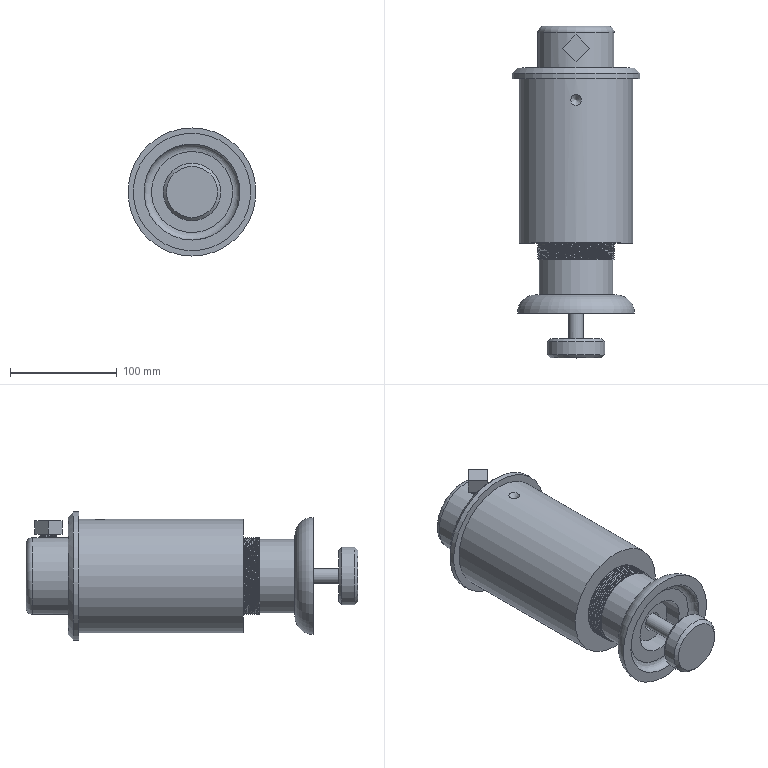Assembly | NX | mm | 5 component files | 5 solids | 128 faces | box 120 x 311 x 120 mm | volume 1746879 mm3 | cylinder 66 | plane 33 | spline 20 | cone 6 | torus 3 | commonest cylinder face diameters 14 x40 72 x4 12 x2 40 x2 45 x2 16 x2 43.5 x2 70 x2
Bill of materials:
unnamed part 1 | 1 |  | Hollow, axially symmetric flanged sleeve. A large flange with a rounded outer edge sits at one end. Next to it is a plain cylindrical section, followed by an externally threaded section that runs to the far end. A through-bore runs along the axis, and the flange face has a shallow stepped recess around the bore.
unnamed part 2 | 1 |  | Thick-walled cylindrical tube with a thin flange at one end. The flange's outer edge is chamfered. There is a small radial hole in the wall near the flange, and the bore at the non-flanged end appears to be internally threaded.
unnamed part 3 | 1 |  | Square-head bolt or screw. It has a square prismatic head and a fully threaded cylindrical shank with a chamfered tip.
unnamed part 4 | 1 |  | Stepped cylindrical shaft or body. The larger-diameter section has a rounded end, a large transverse through-hole, and a small radial hole that appears threaded near the end. The smaller-diameter section has an externally threaded band between plain sections, and an axial bore opens at the small end.
unnamed part 5 | 1 |  | Long slender screw with a short cylindrical head chamfered on both edges. A long plain unthreaded shank leads to an externally threaded section at the tip.
Mates:
1. fix | tool_holder 1 component
2. touch align | bushing 1 face | tool_holder 1 face
3. touch align | screw_sleeve 1 face | bushing 1 face
4. distance | screw_sleeve 1 face | bushing 1 face
5. distance | bushing 1 face | tool_holder 1 face
6. concentric | screw 1 arc | tool_holder 1 arc
7. touch align | screw_rod 1 face | tool_holder 1 face